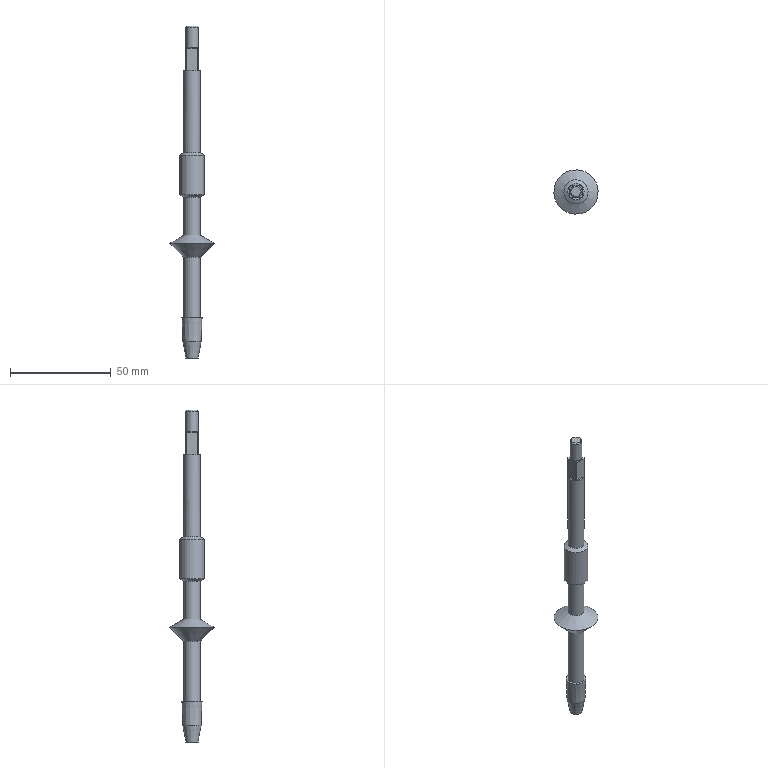Component | NX | VALVE_STEM | 1 solid | 26 faces | volume 10927 mm3 | plane 13 | cone 7 | cylinder 6 | commonest cylinder face diameters 8 x3 12 x1 5 x1 6 x1